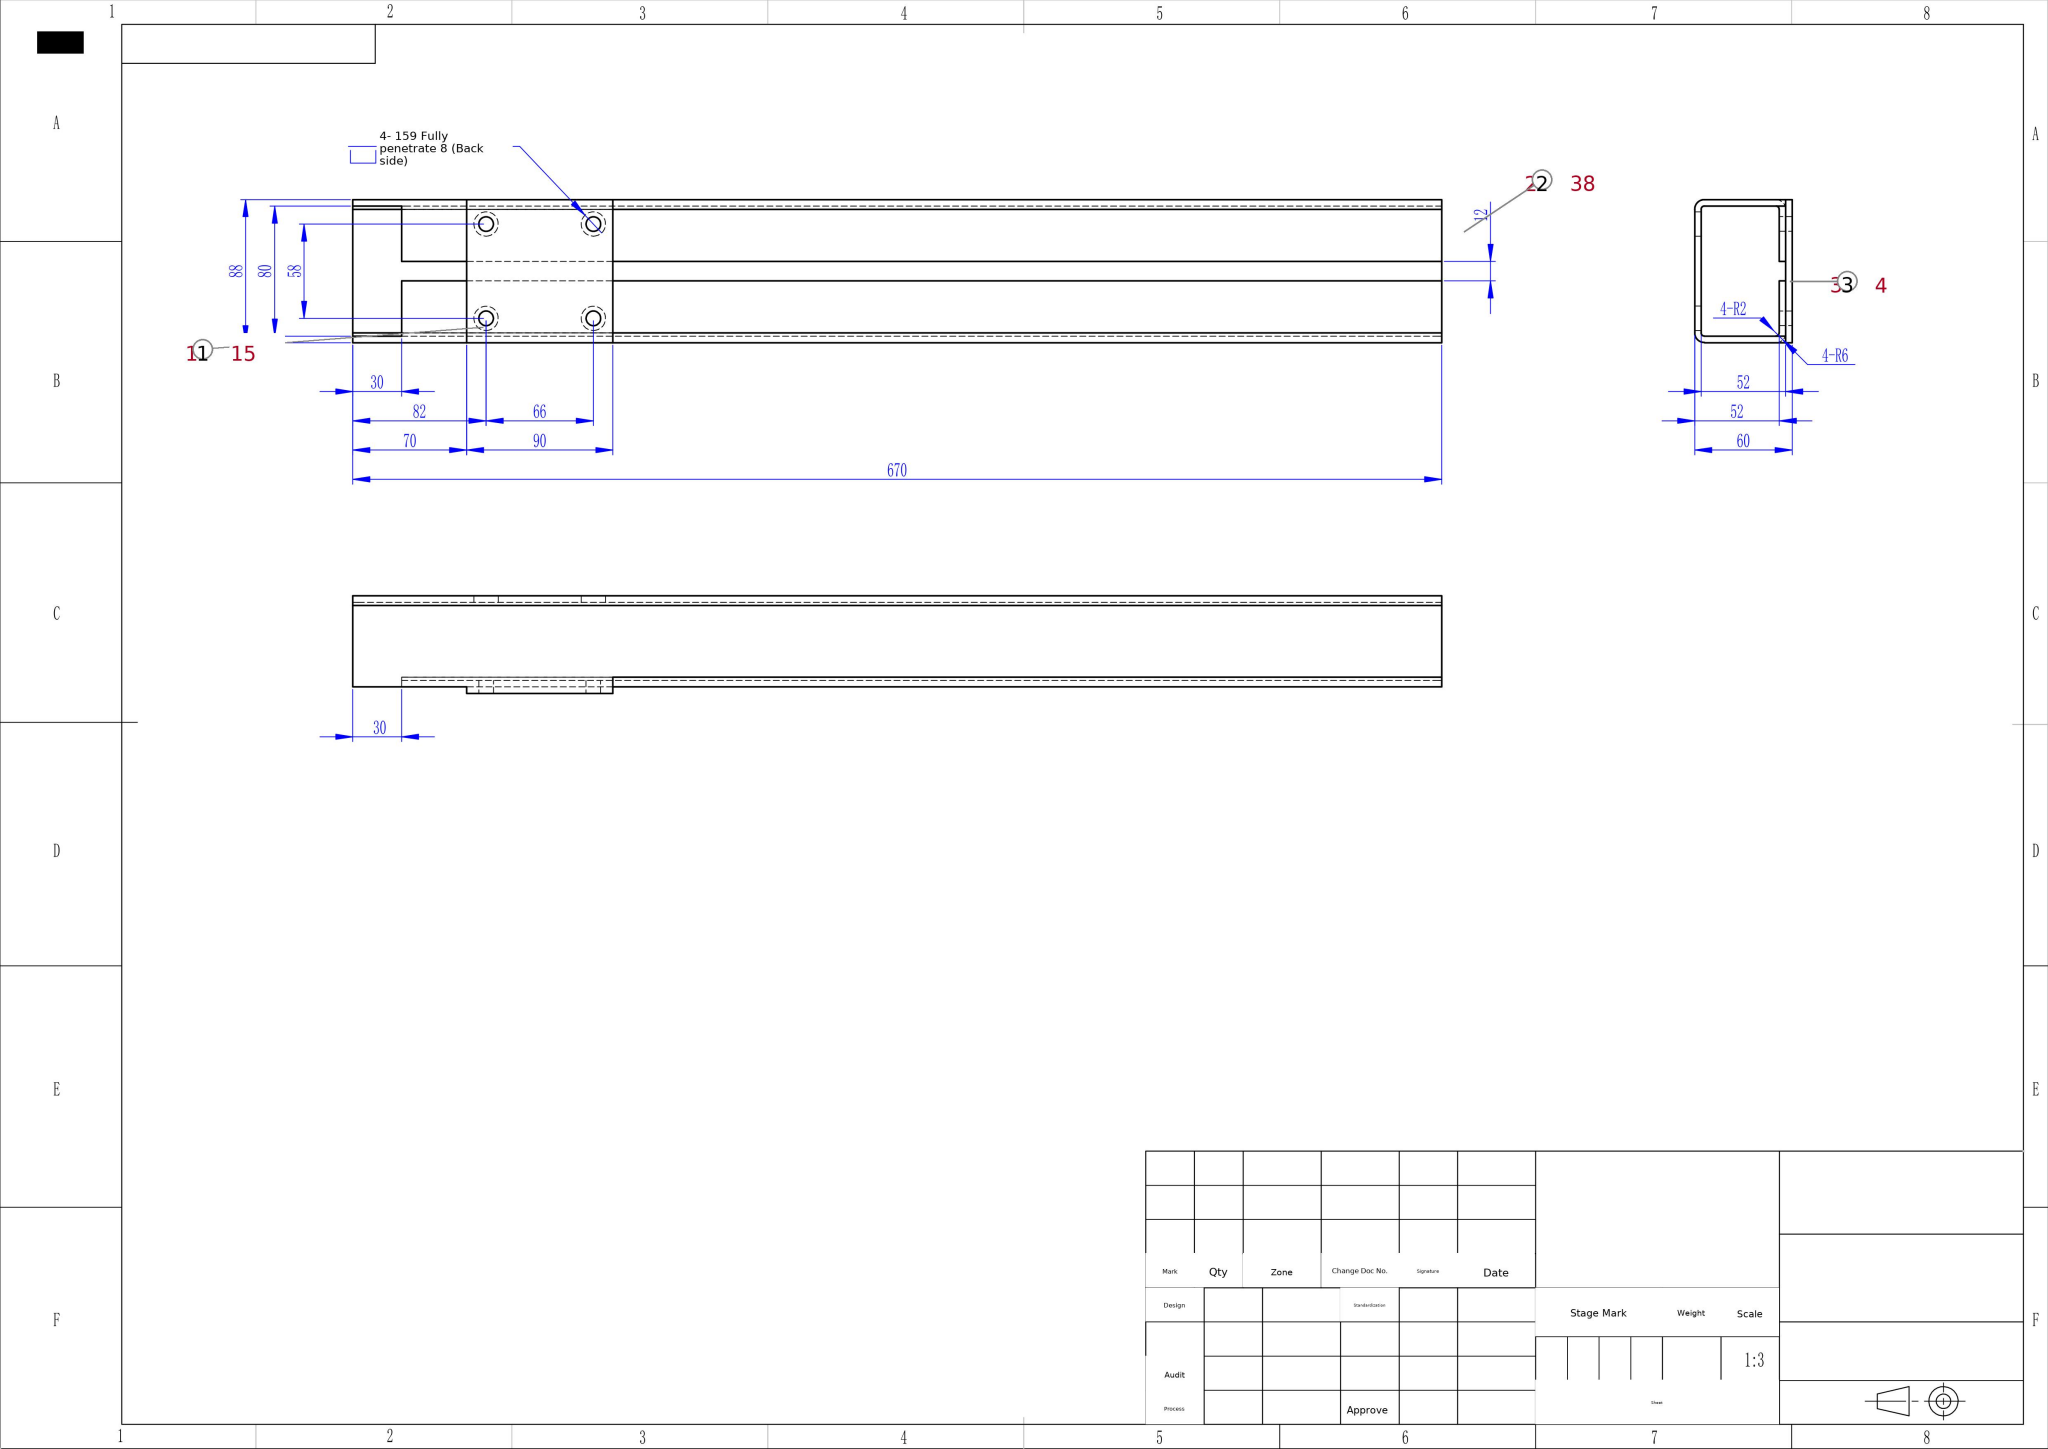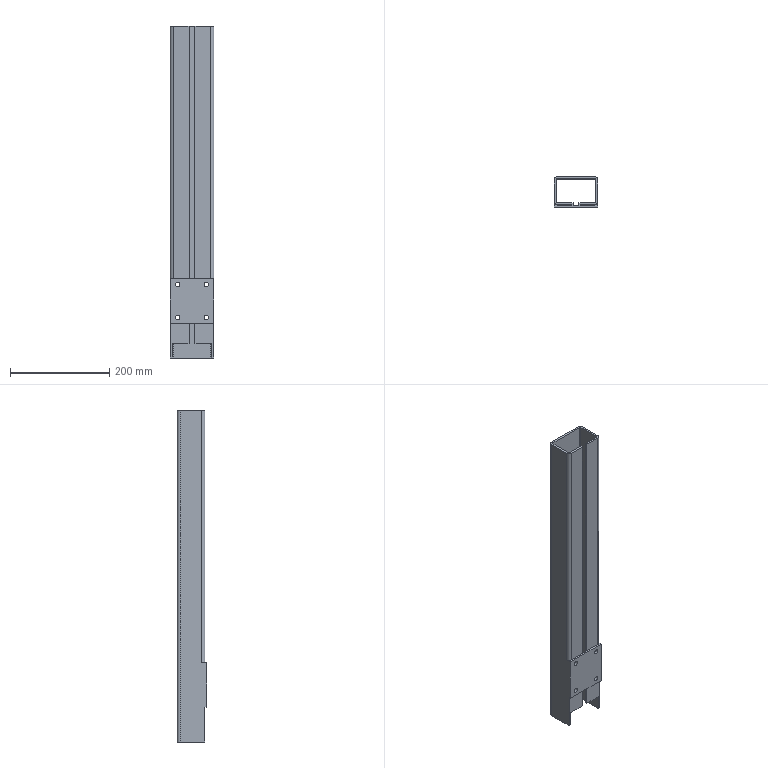Part | SolidWorks | mm | 1 solid | 46 faces | box 88 x 60 x 670 mm | volume 699473 mm3 | cylinder 24 | plane 22 | commonest cylinder face diameters 9 x8 15 x8 4 x4 12 x4
build123d program:
from build123d import *

# Parameters (mm, degrees)
EXTRUDE_THIN1_DEPTH                             = 335
SKETCH2_W                                       = 88
SKETCH2_H                                       = 90
BOSS_EXTRUDE1_DEPTH                             = 4
SKETCH3_W                                       = 80
SKETCH3_H                                       = 30.243
CUT_EXTRUDE1_DEPTH                              = 10
FILLET1_R                                       = 2
FILLET2_R                                       = 6
M8_HEX_SOCKET_HEAD_CAP_SCREW_CBORE1_D           = 9
M8_HEX_SOCKET_HEAD_CAP_SCREW_CBORE1_CBORE_D     = 15
M8_HEX_SOCKET_HEAD_CAP_SCREW_CBORE1_CBORE_DEPTH = 8


with BuildPart() as part:
    # Sketch1 → Extrude-Thin1 (new, symmetric)
    with BuildSketch(Plane.XY):
        Polygon((6, -24), (40, -24), (40, 24), (-40, 24), (-40, -24), (-6, -24), (-6, -28), (-44, -28), (-44, 28), (44, 28), (44, -28), (6, -28), align=None)
    extrude(amount=EXTRUDE_THIN1_DEPTH, both=True)

    # Sketch2 → Boss-Extrude1 (add)
    with BuildSketch(Plane.XZ.offset(28)):
        with Locations((0, -220)):
            Rectangle(SKETCH2_W, SKETCH2_H)
    extrude(amount=BOSS_EXTRUDE1_DEPTH)

    # Sketch3 → Cut-Extrude1 (cut)
    with BuildSketch(Plane.XZ.offset(28)):
        with Locations((0, -320.122)):
            Rectangle(SKETCH3_W, SKETCH3_H)
    extrude(amount=-CUT_EXTRUDE1_DEPTH, mode=Mode.SUBTRACT)

    # Fillet1
    fillet1_edges = [part.edges().sort_by_distance(p)[0] for p in [
        (40, -24, 15),
        (40, 24, 0),
        (-40, 24, 0),
        (-40, -24, 15),
    ]]
    fillet(fillet1_edges, radius=FILLET1_R)

    # Fillet2
    fillet2_edges = [part.edges().sort_by_distance(p)[0] for p in [
        (-44, -28, 80),
        (-44, 28, 0),
        (44, 28, 0),
        (44, -28, 80),
    ]]
    fillet(fillet2_edges, radius=FILLET2_R)

    # M8 Hex Socket Head Cap Screw CBORE1 (through all)
    with Locations(Plane(origin=(0, 28, 0), x_dir=(-1, 0, 0), z_dir=(0, 1, 0))):
        with Locations((-29, -187), (-29, -253), (29, -253), (29, -187)):
            CounterBoreHole(M8_HEX_SOCKET_HEAD_CAP_SCREW_CBORE1_D / 2, M8_HEX_SOCKET_HEAD_CAP_SCREW_CBORE1_CBORE_D / 2, M8_HEX_SOCKET_HEAD_CAP_SCREW_CBORE1_CBORE_DEPTH)


solid = part.part